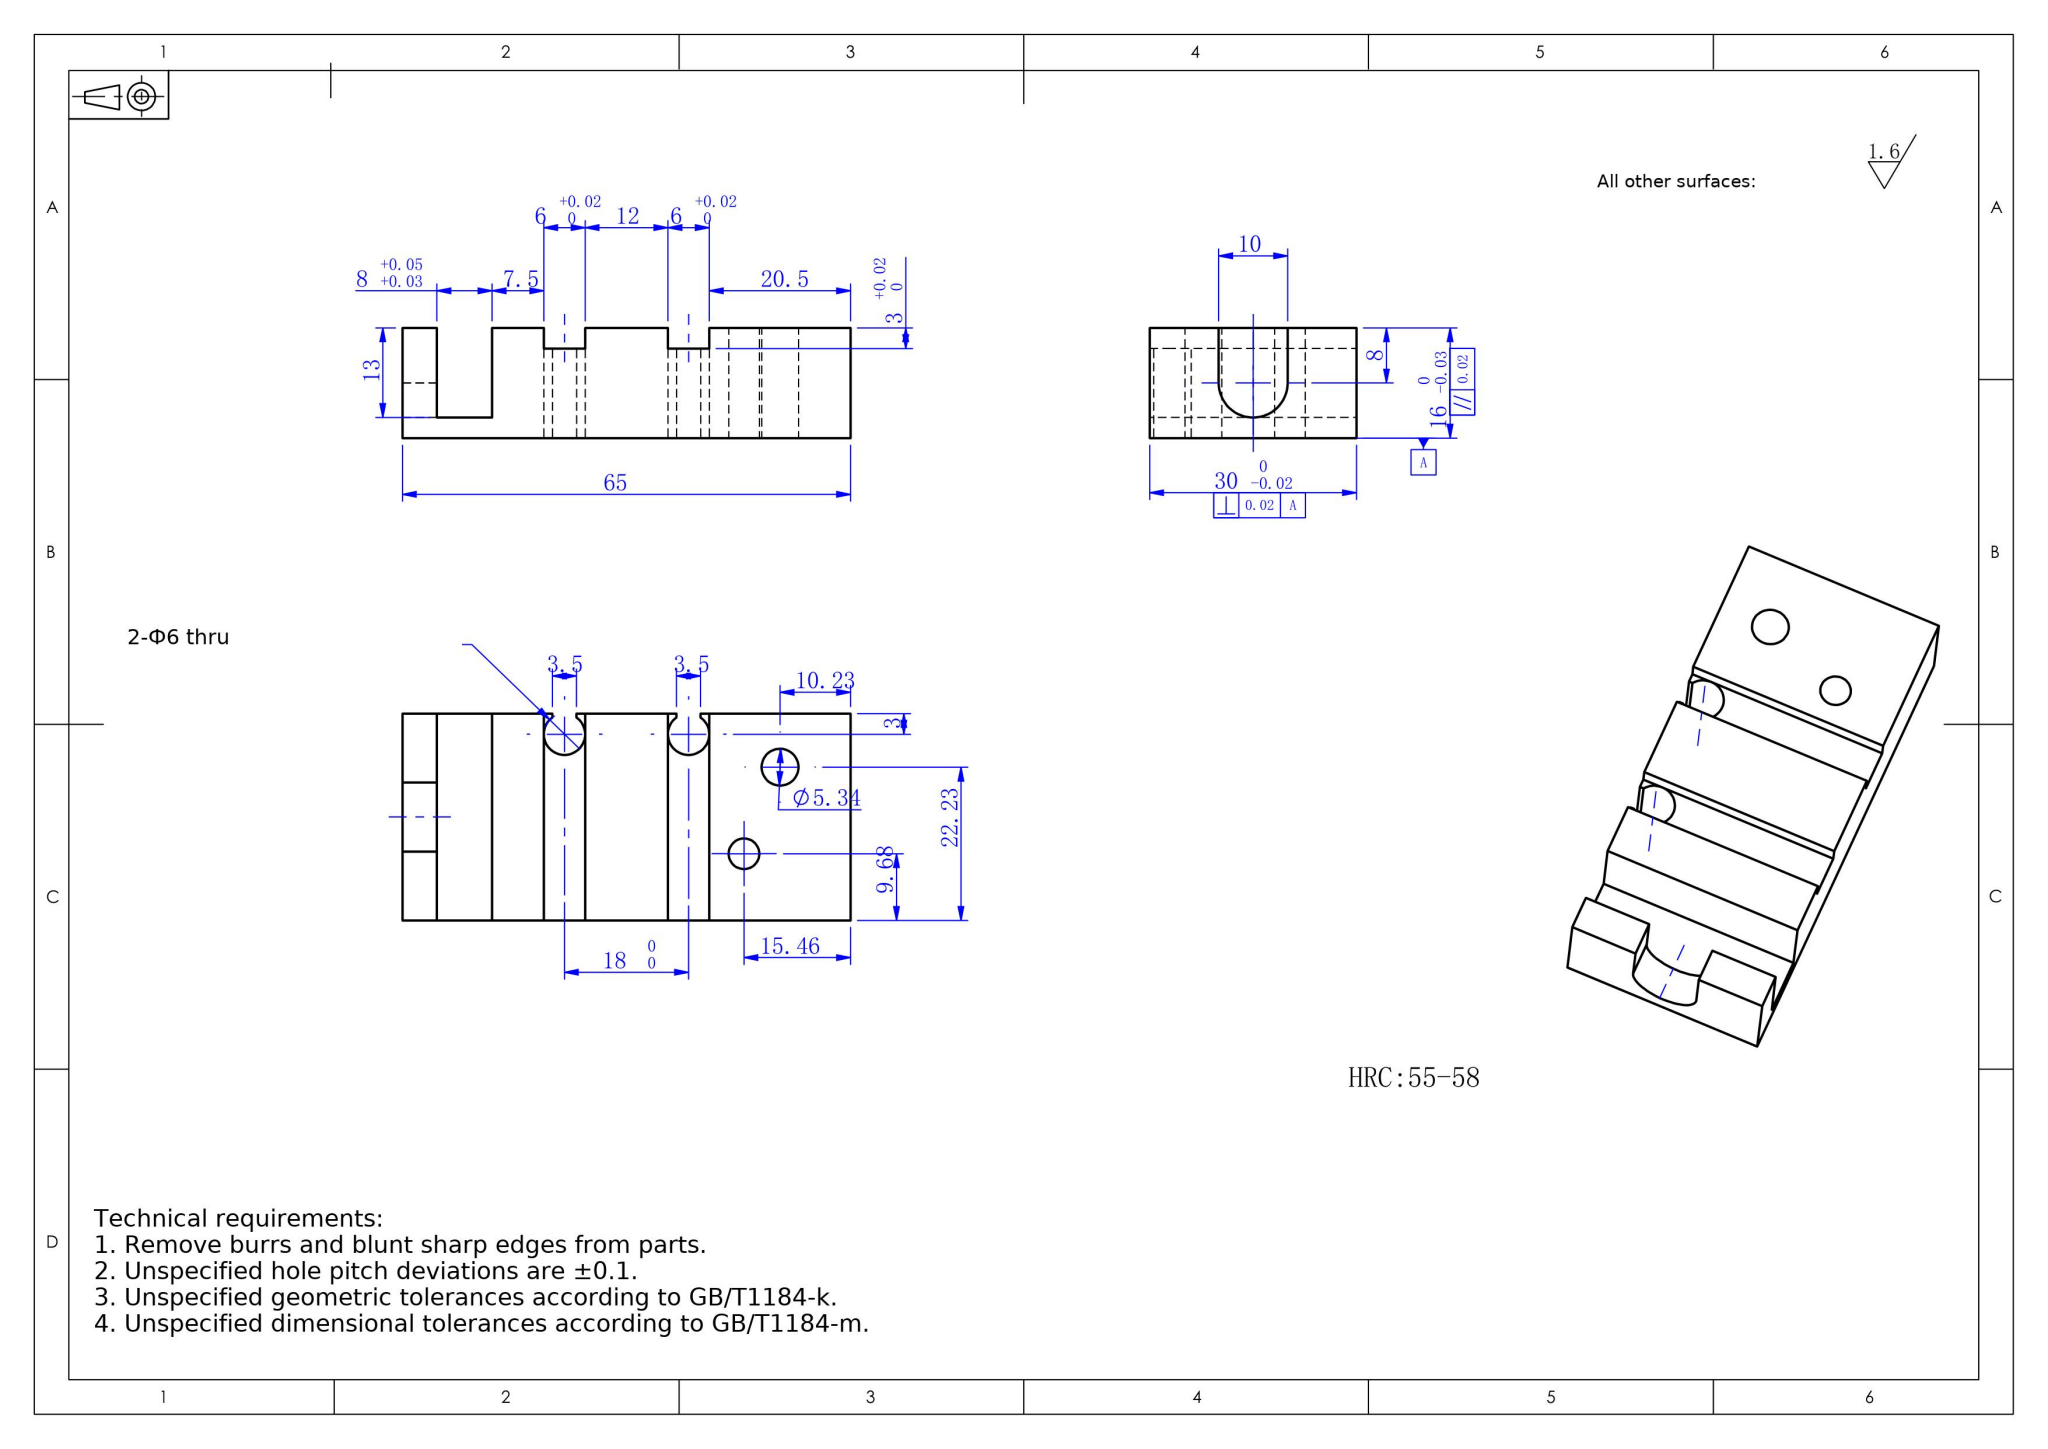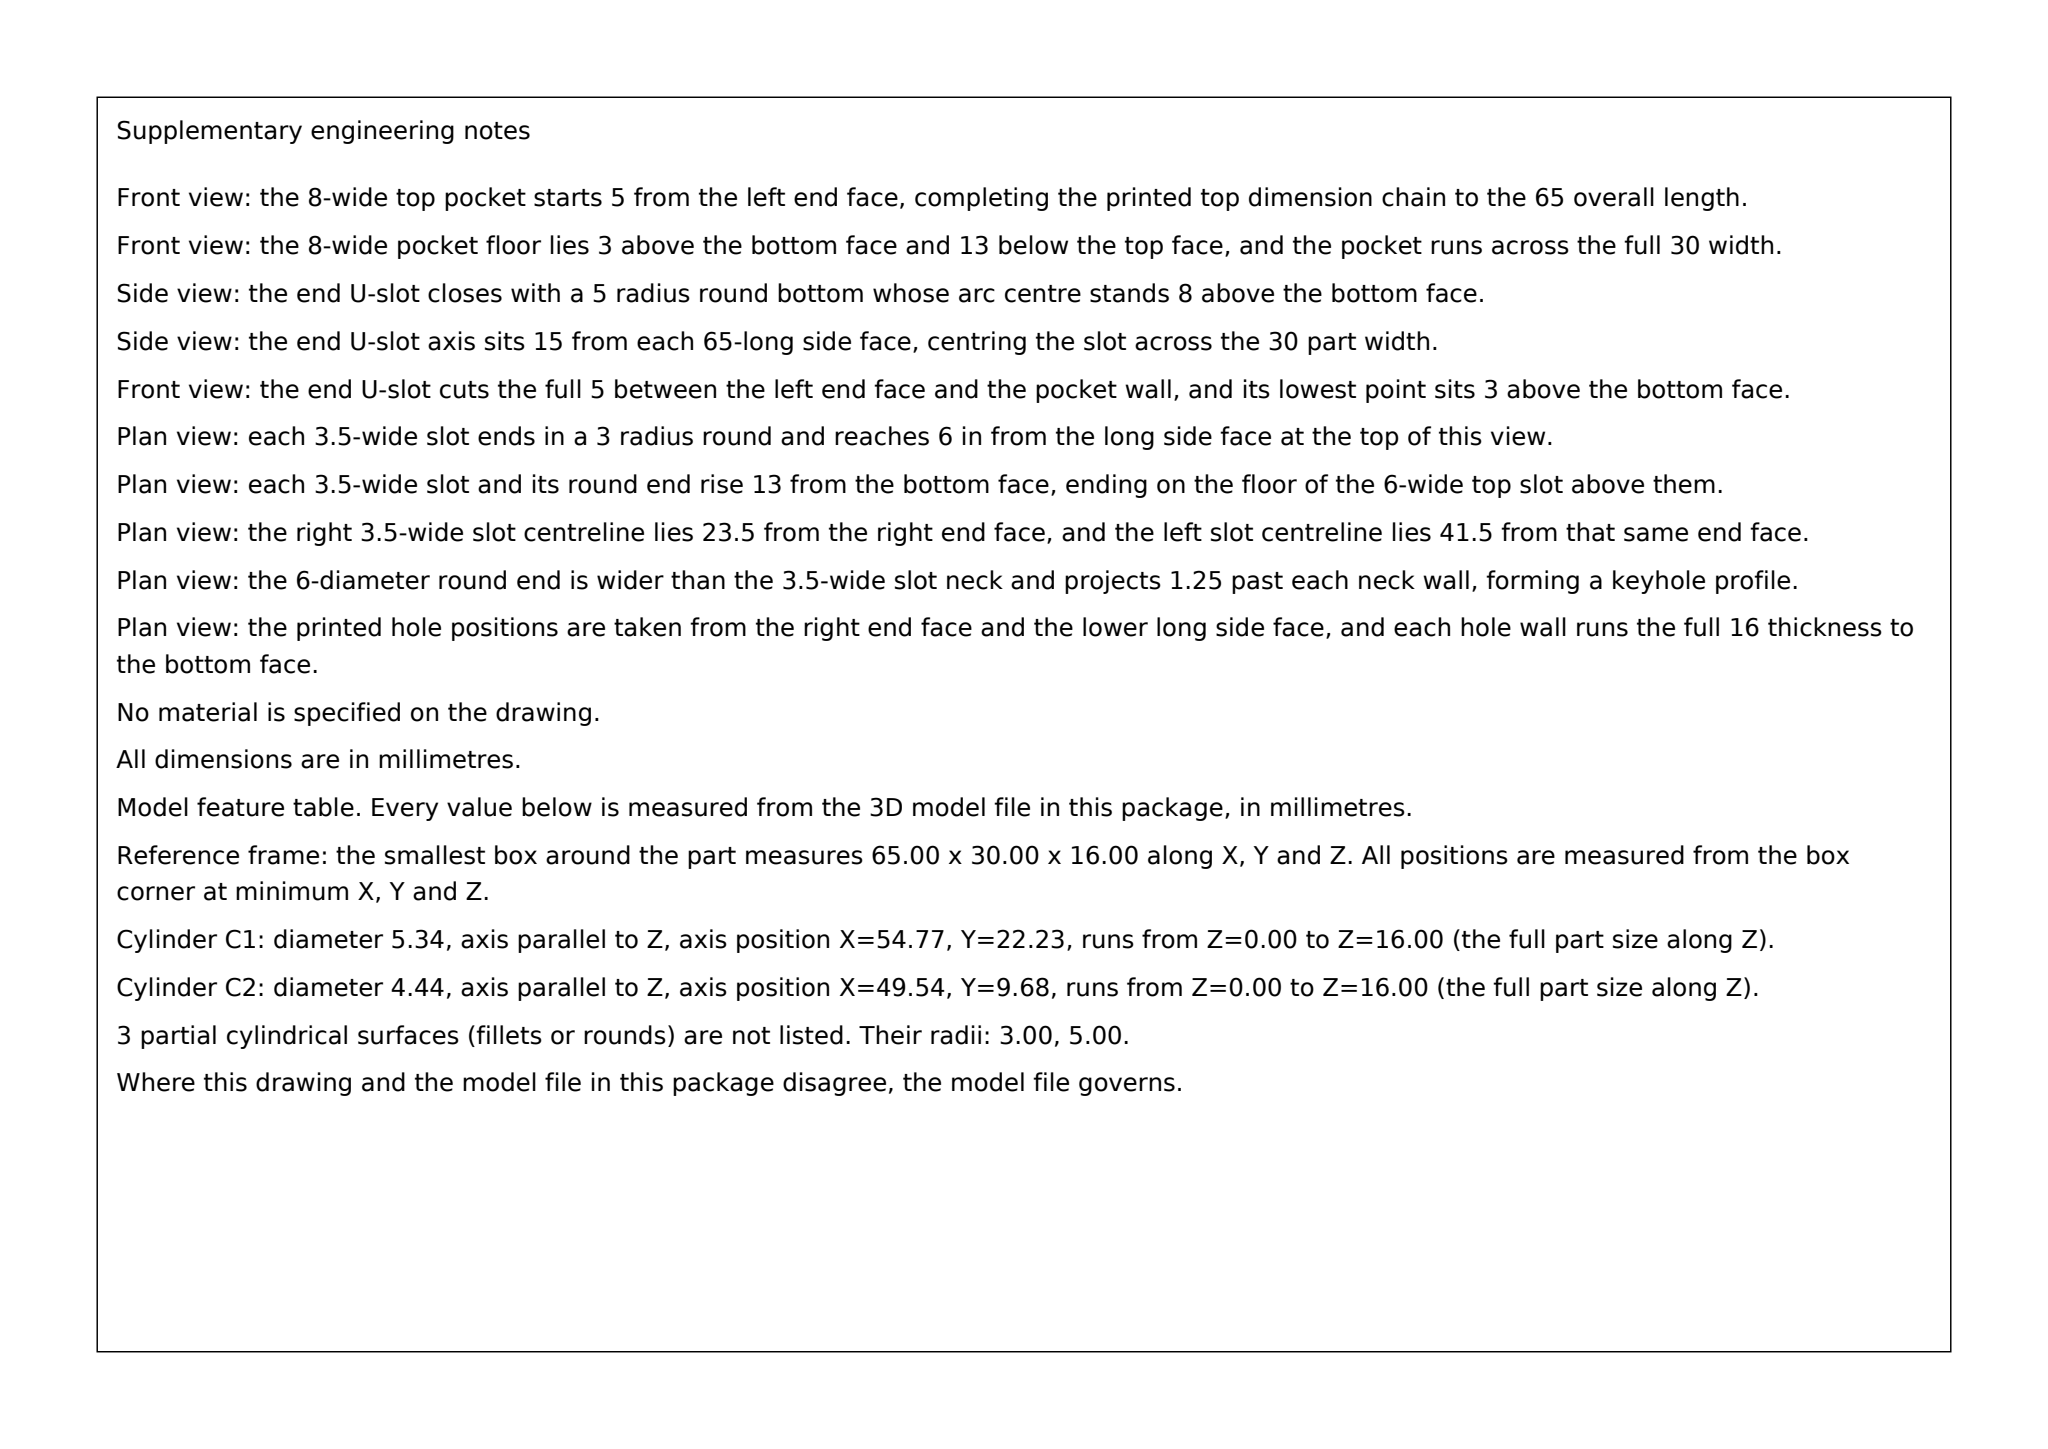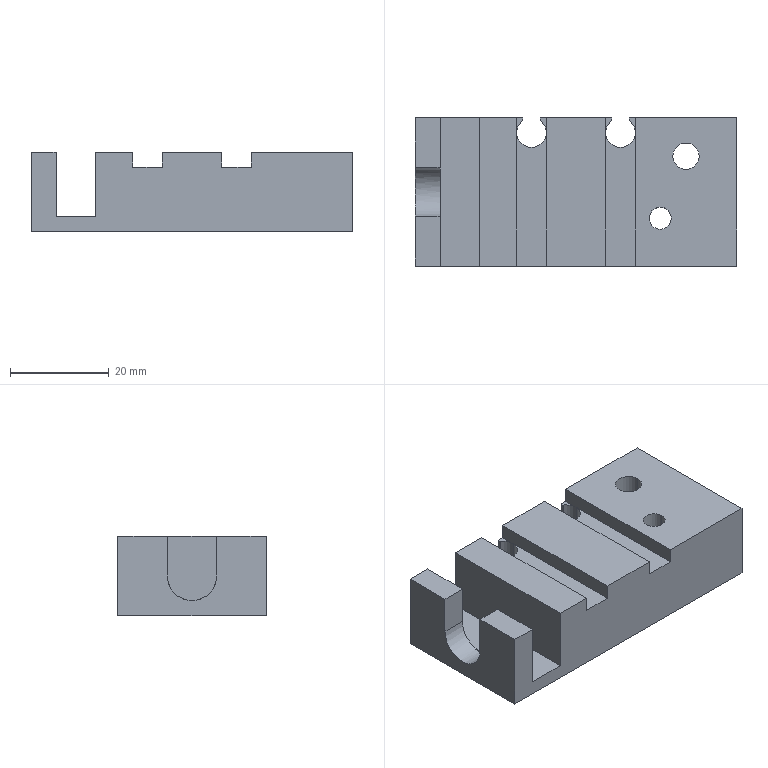Part | SolidWorks | mm | 1 solid | 43 faces | box 65 x 30 x 16 mm | volume 25046 mm3 | plane 32 | cylinder 11 | commonest cylinder face diameters 6 x6 5.34 x2 4.438 x2 10 x1
Drawing notes:
2ND HOLE (15.46 & 9.68 FROM EDGES): Ø4.438 THRU | from the solid: cylinder dia 4.438, axis z, pos (49.54, 9.68), length 16 = full 16 thk (thru)
2-3.5 WIDE SLOTS W/ Ø6 ROUND END: 13 DEEP FROM TOP FACE | from the solid: cylinders dia 6.0, axis z at x=23.5 & 41.5, y=27, length 13 from z=16 top face down to z=3
10 WIDE ROUND-END SLOT IN LEFT END FACE: 5 DEEP (X 0 TO 5) | from the solid: cylinder dia 10, axis x, pos y=15 z=8, length 5; x-planes at 0.0 and 5.0
2X 3.5 WIDE SLOT (Ø6 ROUND END, 13 DEEP FROM TOP FACE): SLOT CENTRELINES LOCATED 23.5 AND 41.5 FROM LEFT END FACE (X=0); ROUND-END CENTRES 3 FROM REAR FACE (Y=27 FROM Y=0 FACE) | from the solid: cylinders dia 6, axis z, pos (23.5,27) and (41.5,27), length 13; axis_planes x=21.75/25.25 and x=39.75/43.25 (3.5 wide slot walls)
2X 3.5 WIDE SLOT (Ø6 ROUND END, 13 DEEP FROM TOP FACE): SLOT CENTRELINES AT 23.5 AND 41.5 FROM LEFT END FACE (X=0); ROUND-END CENTRES AT 27 FROM FRONT FACE (Y=0) | from the solid: cylinders dia 6.0, axis z, positions (23.5, 27.0) and (41.5, 27.0), length 13.0; bbox 65 x 30 x 16
build123d program:
from build123d import *

# Parameters (mm, degrees)
BOSS_EXTRUDE1_DEPTH = 16
SKETCH2_W           = 6
SKETCH2_H           = 30
CUT_EXTRUDE1_DEPTH  = 3
SKETCH7_W           = 8
SKETCH7_H           = 13
CUT_EXTRUDE8_DEPTH  = 71.273
CUT_EXTRUDE9_REACH  = 86.155
SKETCH9_R           = 2.67
SKETCH9_R_2         = 2.219
CUT_EXTRUDE10_DEPTH = 80


with BuildPart() as part:
    # Sketch1 → Boss-Extrude1 (new body)
    with BuildSketch(Plane.XY):
        with BuildLine():
            Line((-61.5, -21), (-39.75, -21))
            Line((-39.75, -21), (-39.75, -21.563))
            ThreePointArc((-39.75, -21.563), (-38, -27), (-36.25, -21.563))
            Line((-36.25, -21.563), (-36.25, -21))
            Line((-36.25, -21), (-21.75, -21))
            Line((-21.75, -21), (-21.75, -21.563))
            ThreePointArc((-21.75, -21.563), (-20, -27), (-18.25, -21.563))
            Line((-18.25, -21.563), (-18.25, -21))
            Line((-18.25, -21), (3.5, -21))
            Line((3.5, -21), (3.5, -51))
            Line((3.5, -51), (-61.5, -51))
            Line((-61.5, -51), (-61.5, -21))
        make_face()
    extrude(amount=BOSS_EXTRUDE1_DEPTH)

    # Sketch2 → Cut-Extrude1 (cut)
    with BuildSketch(Plane.XY.offset(16)):
        with Locations((-20, -36)):
            Rectangle(SKETCH2_W, SKETCH2_H)
        with Locations((-38, -36)):
            Rectangle(SKETCH2_W, SKETCH2_H)
    extrude(amount=-CUT_EXTRUDE1_DEPTH, mode=Mode.SUBTRACT)

    # Sketch7 → Cut-Extrude8 (cut, through all)
    with BuildSketch(Plane(origin=(0, -51, 0), x_dir=(-1, 0, 0), z_dir=(0, -1, 0))):
        with Locations((52.5, -9.5)):
            Rectangle(SKETCH7_W, SKETCH7_H)
    extrude(amount=-CUT_EXTRUDE8_DEPTH, mode=Mode.SUBTRACT)

    # Sketch8 → Cut-Extrude9 (cut, up to next)
    with BuildSketch(Plane.ZY.offset(61.5), mode=Mode.PRIVATE) as cut_extrude9_sk1:
        with BuildLine():
            Line((8, -31), (16, -31))
            Line((16, -31), (16, -41))
            Line((16, -41), (8, -41))
            ThreePointArc((8, -41), (3, -36), (8, -31))
        make_face()
    cut_extrude9_tool1 = extrude(cut_extrude9_sk1.sketch, amount=-CUT_EXTRUDE9_REACH, mode=Mode.PRIVATE) & part.part
    add(cut_extrude9_tool1.solids().sort_by_distance((-61.5, -36, 9.984))[0], mode=Mode.SUBTRACT)

    # Sketch9 → Cut-Extrude10 (cut)
    with BuildSketch(Plane.XY.offset(16)):
        with Locations((-6.734, -28.77)):
            Circle(SKETCH9_R)
        with Locations((-11.964, -41.323)):
            Circle(SKETCH9_R_2)
    extrude(amount=-CUT_EXTRUDE10_DEPTH, mode=Mode.SUBTRACT)


solid = part.part